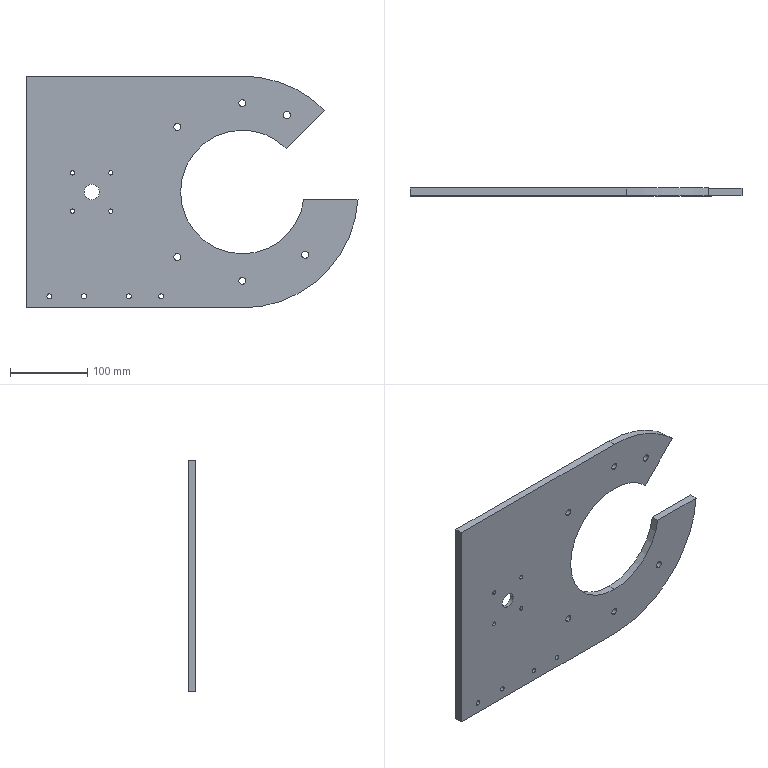Component | SolidWorks | FixedPlate-1 | 1 solid | 65 faces | volume 903849 mm3 | cylinder 37 | cone 20 | plane 8 | commonest cylinder face diameters 9 x12 6.5 x8 5.5 x8 160 x3 52 x2 20 x2 300 x2